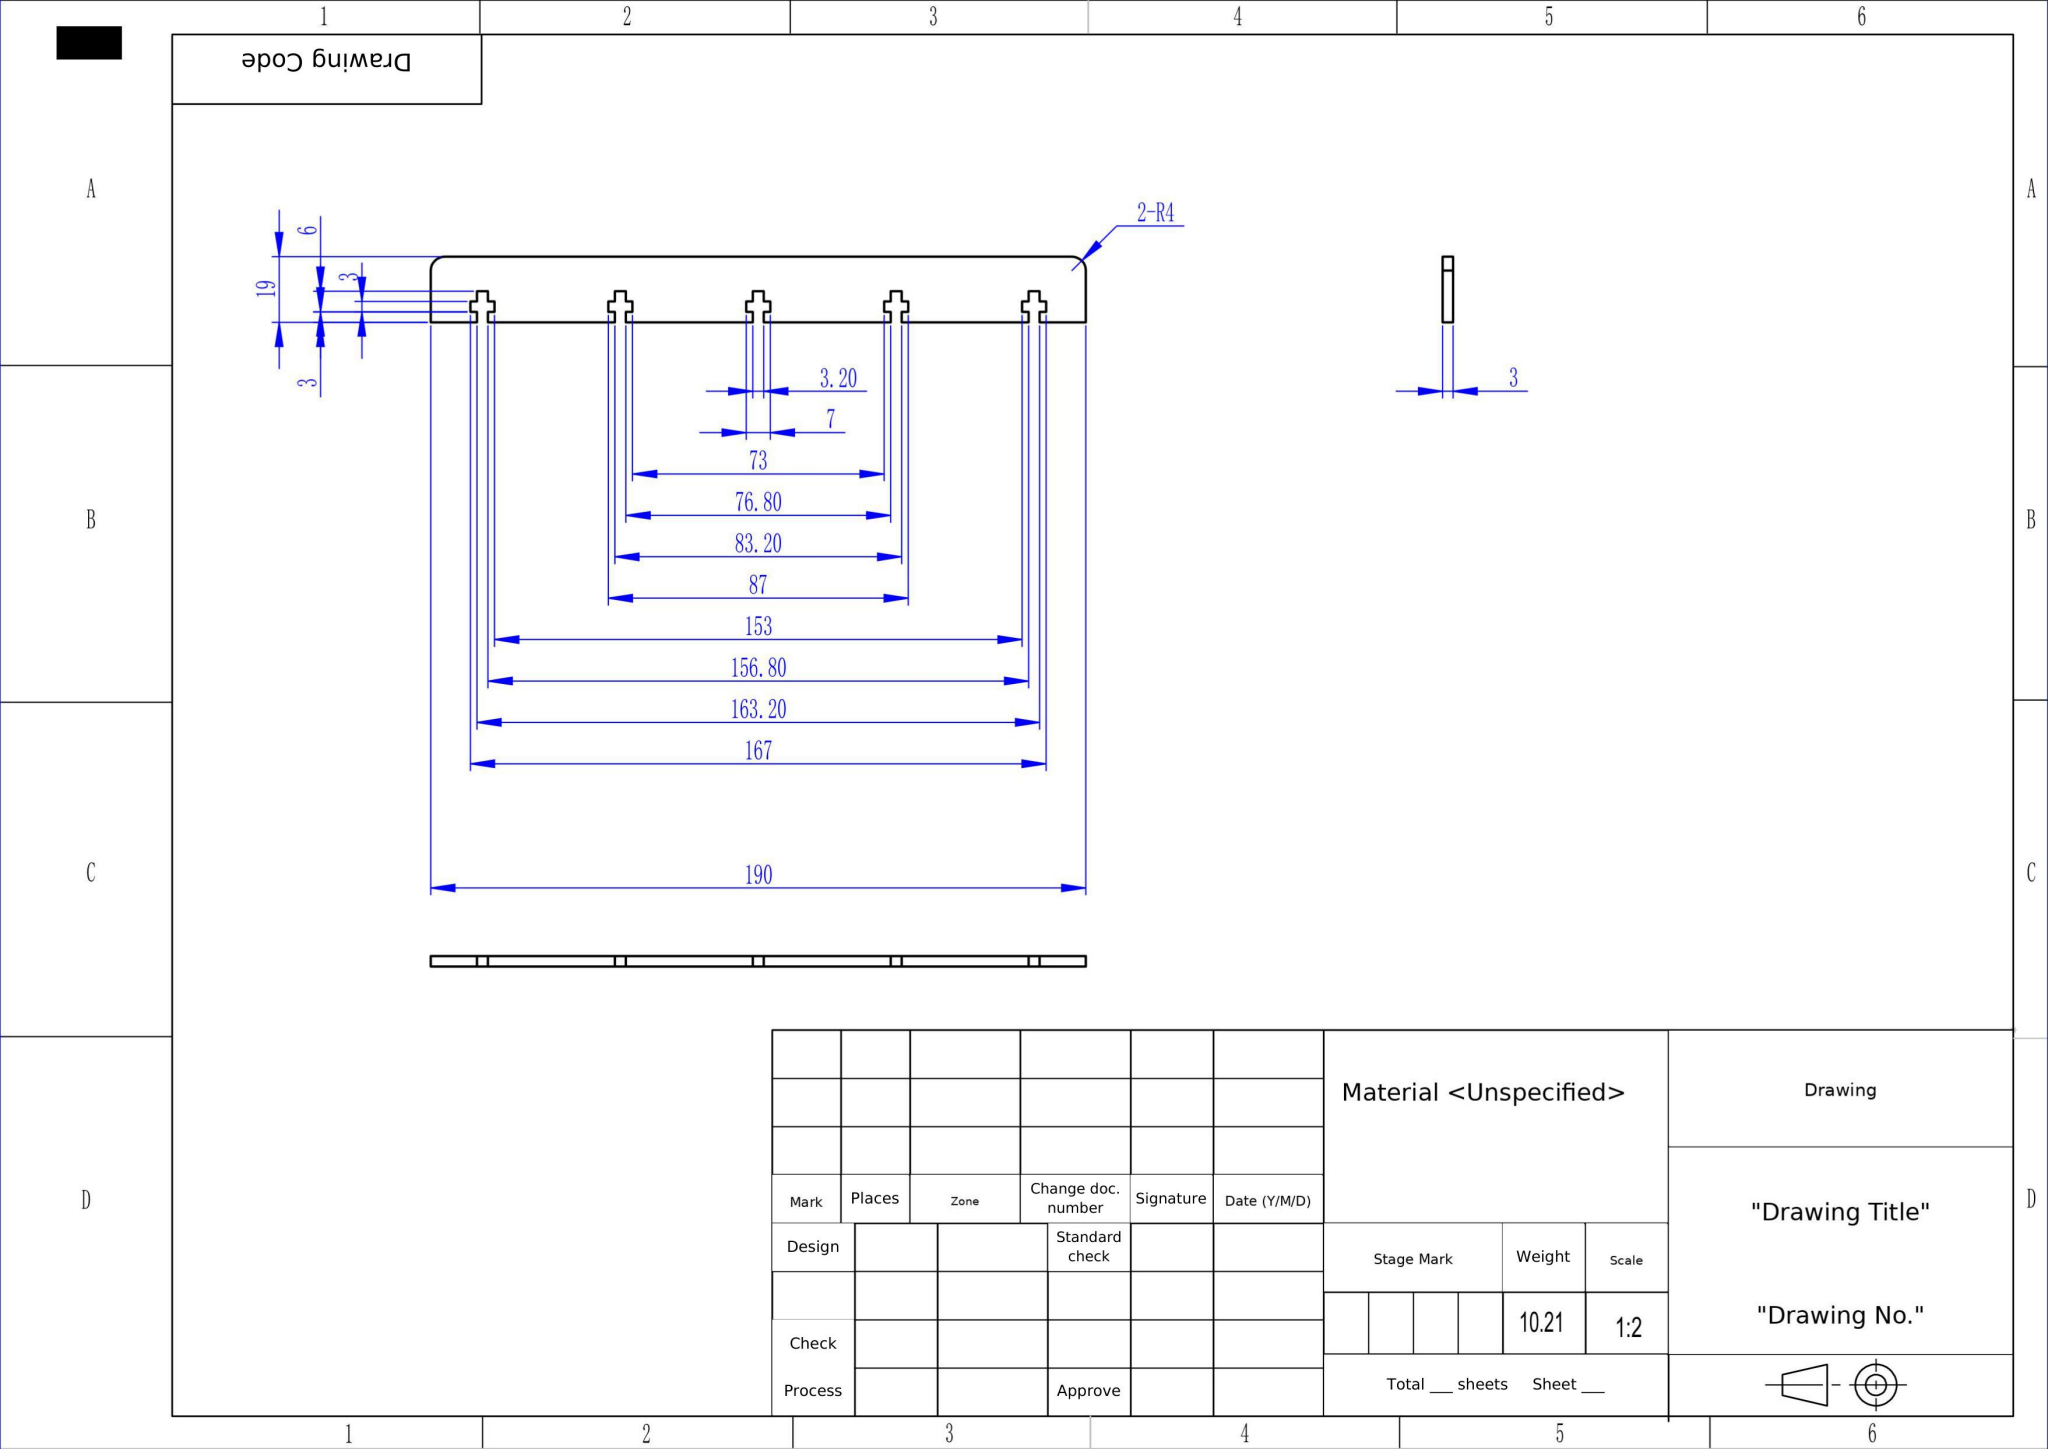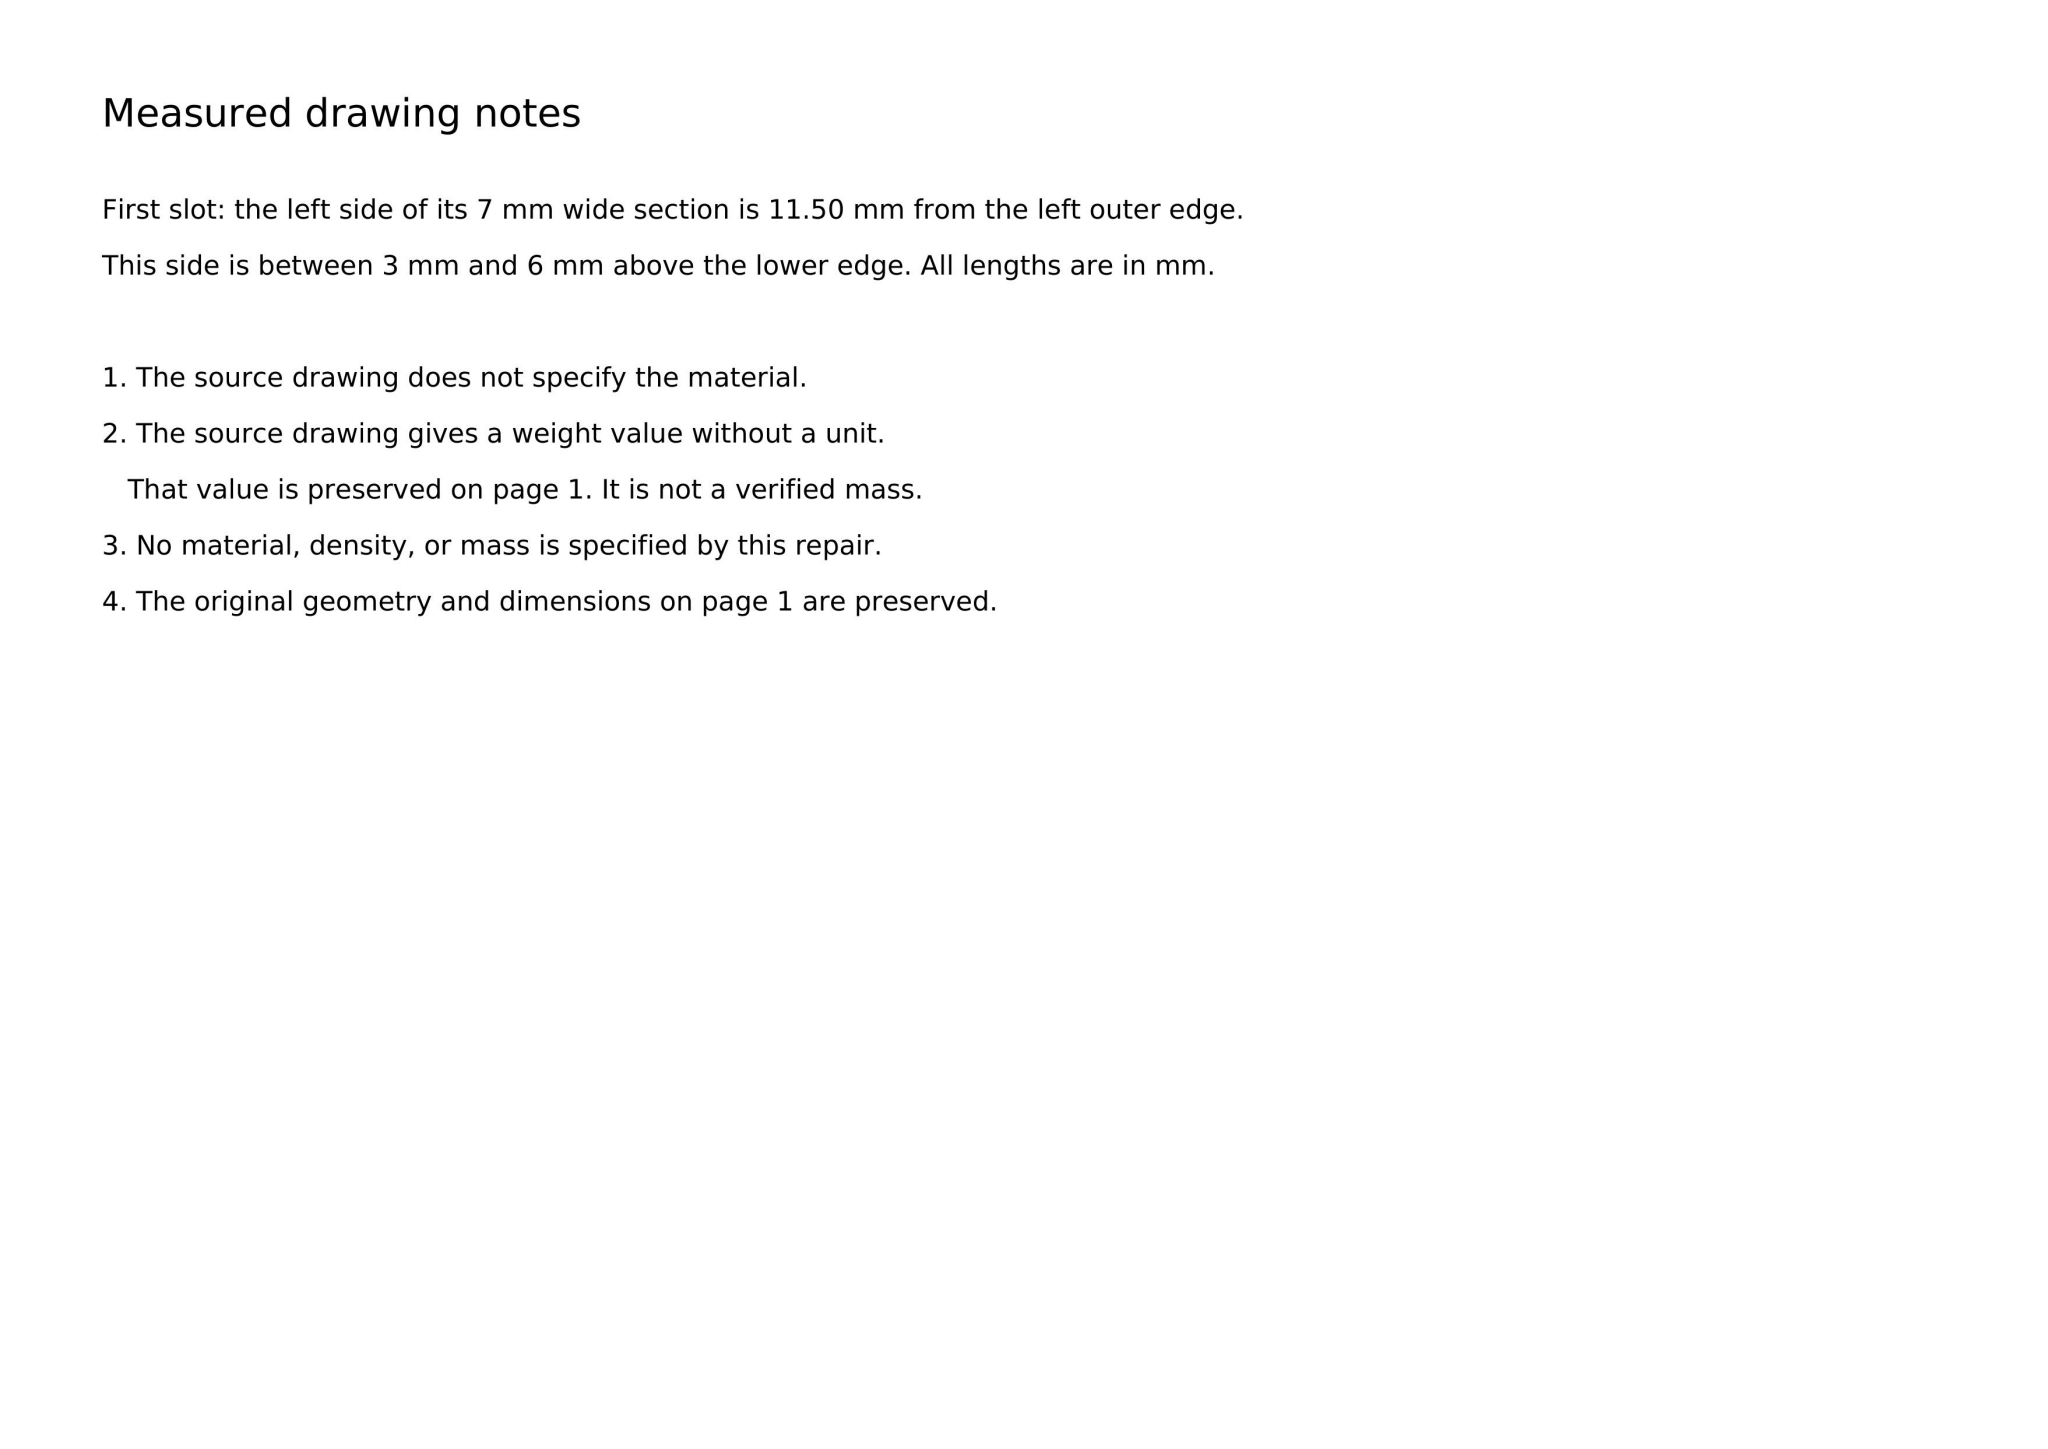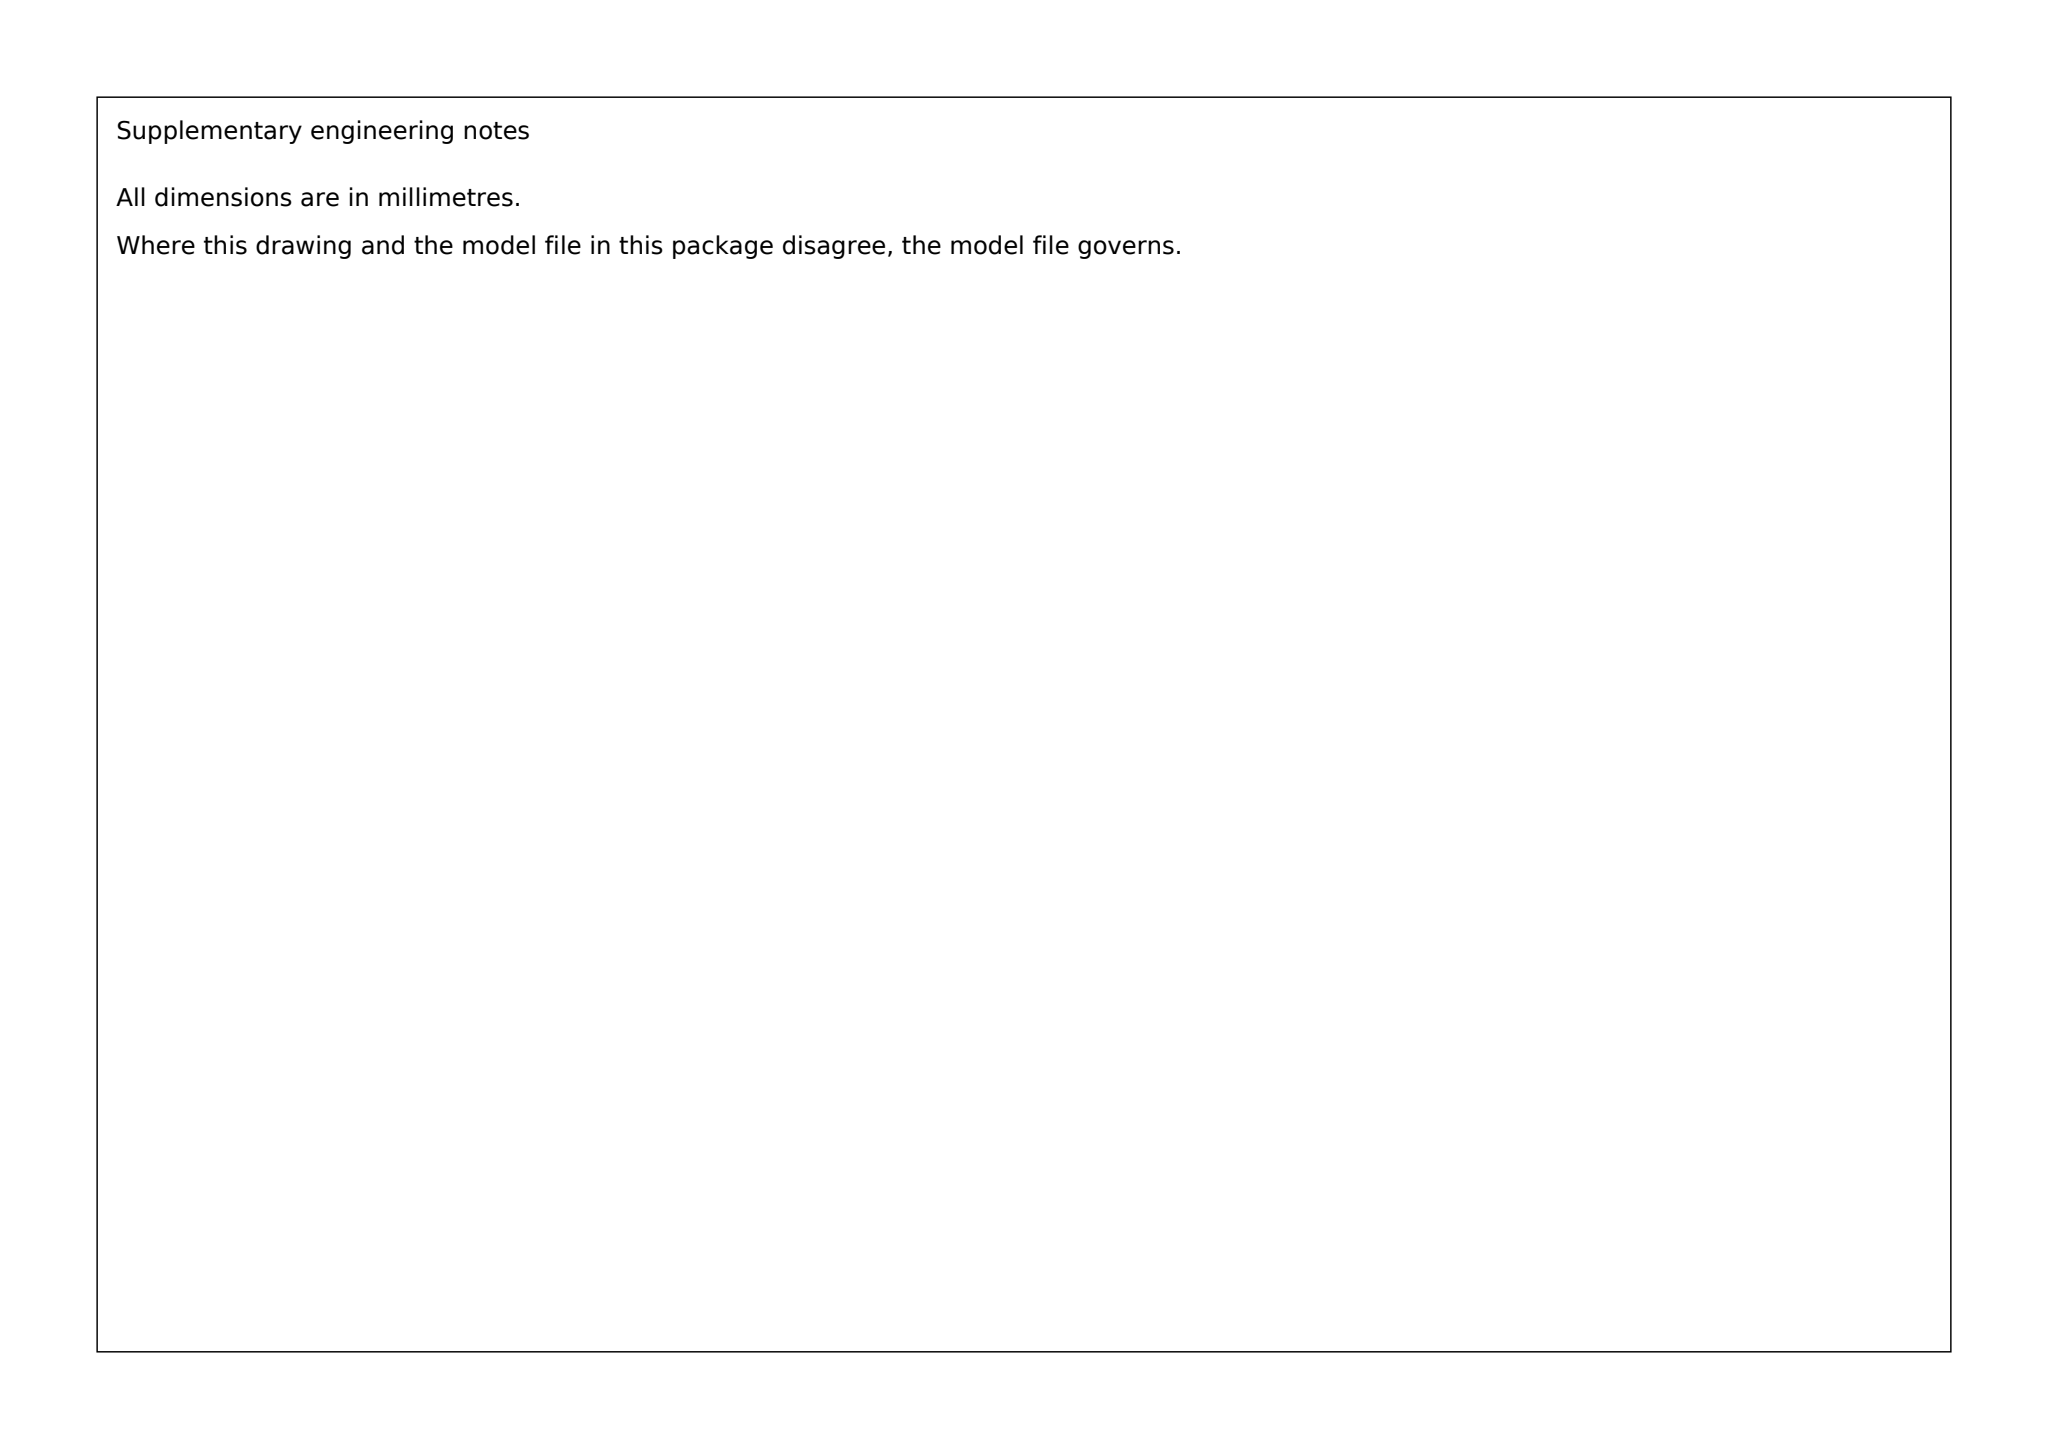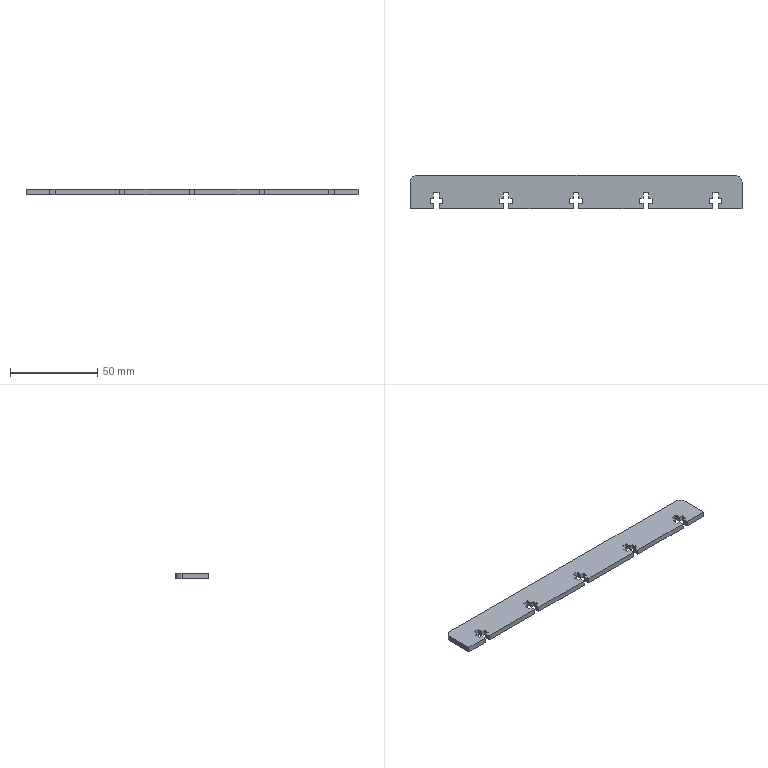Part | SolidWorks | mm | 1 solid | 68 faces | box 190 x 19 x 3 mm | volume 10206 mm3 | plane 66 | cylinder 2 | commonest cylinder face diameters 8 x2
build123d program:
from build123d import *

# Parameters (mm, degrees)
BOSS_EXTRUDE1_DEPTH = 3
FILLET1_R           = 4


with BuildPart() as part:
    # Sketch1 → Boss-Extrude1 (new body)
    with BuildSketch(Plane.XY):
        Polygon((13.4, 0), (13.4, 3), (11.5, 3), (11.5, 6), (13.4, 6), (13.4, 9), (16.6, 9), (16.6, 6), (18.5, 6), (18.5, 3), (16.6, 3), (16.6, 0), (53.4, 0), (53.4, 3), (51.5, 3), (51.5, 6), (53.4, 6), (53.4, 9), (56.6, 9), (56.6, 6), (58.5, 6), (58.5, 3), (56.6, 3), (56.6, 0), (93.4, 0), (93.4, 3), (91.5, 3), (91.5, 6), (93.4, 6), (93.4, 9), (96.6, 9), (96.6, 6), (98.5, 6), (98.5, 3), (96.6, 3), (96.6, 0), (133.4, 0), (133.4, 3), (131.5, 3), (131.5, 6), (133.4, 6), (133.4, 9), (136.6, 9), (136.6, 6), (138.5, 6), (138.5, 3), (136.6, 3), (136.6, 0), (163.2, 0), (170.7, 0), (173.4, 0), (173.4, 3), (171.5, 3), (171.5, 6), (173.4, 6), (173.4, 9), (176.6, 9), (176.6, 6), (178.5, 6), (178.5, 3), (176.6, 3), (176.6, 0), (190, 0), (190, 19), (0, 19), (0, 0), align=None)
    extrude(amount=BOSS_EXTRUDE1_DEPTH)

    # Fillet1
    fillet1_edges = [part.edges().sort_by_distance(p)[0] for p in [
        (0, 19, 1.5),
        (190, 19, 1.5),
    ]]
    fillet(fillet1_edges, radius=FILLET1_R)


solid = part.part